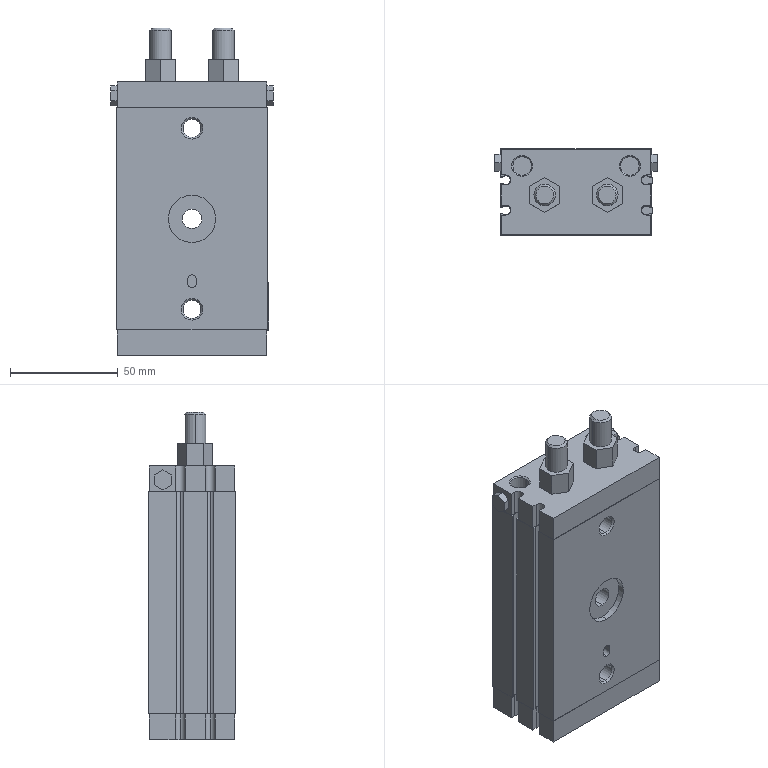Component | SolidWorks | Inline-H010-A_EMSQA30A-A96(0)-1_Inline-H010-1-1 | 1 solid | 204 faces | volume 341159 mm3 | plane 112 | cylinder 64 | cone 28 | commonest cylinder face diameters 4.6 x12 4 x10 4.917 x8 4.2 x6 14 x4 8.6 x4 8.376 x4 2.7 x4